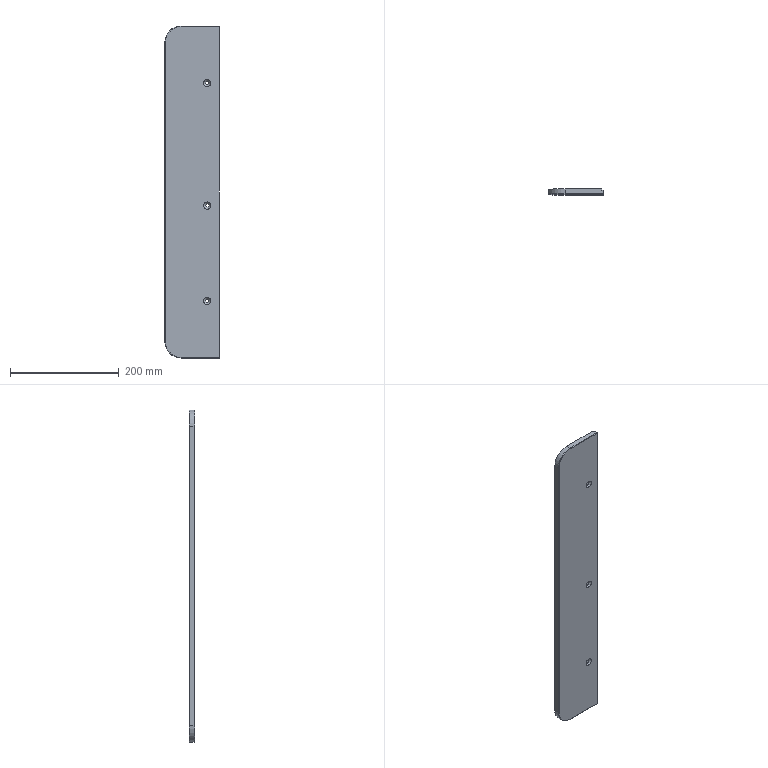Component | SolidWorks | ChainPartTablePlate-1 | 1 solid | 27 faces | box 100 x 10 x 610 mm | volume 601377 mm3 | cylinder 11 | plane 8 | cone 6 | torus 2 | commonest cylinder face diameters 6.6 x6 2 x3 60 x2
build123d program:
from build123d import *

# Parameters (mm, degrees)
SKETCH1_W                                            = 610
SKETCH1_H                                            = 100
BOSS_EXTRUDE1_DEPTH                                  = 10
FILLET1_R                                            = 30
CSK_FOR_M6_HEX_SOCKET_COUNTERSUNK_CAP_SC_D           = 6.6
CSK_FOR_M6_HEX_SOCKET_COUNTERSUNK_CAP_SC_CSINK_D     = 13.6
CSK_FOR_M6_HEX_SOCKET_COUNTERSUNK_CAP_SC_CSINK_ANGLE = 90
SKETCH4_W                                            = 610
SKETCH4_H                                            = 2.5
CUT_EXTRUDE1_DEPTH                                   = 2
FILLET4_R                                            = 1


with BuildPart() as part:
    # Sketch1 → Boss-Extrude1 (new body)
    with BuildSketch(Plane.XY):
        Rectangle(SKETCH1_W, SKETCH1_H)
    extrude(amount=BOSS_EXTRUDE1_DEPTH)

    # Fillet1
    fillet1_edges = [part.edges().sort_by_distance(p)[0] for p in [
        (305, -50, 5),
        (-305, -50, 5),
    ]]
    fillet(fillet1_edges, radius=FILLET1_R)

    # CSK for M6 Hex Socket Countersunk Cap Sc (through all)
    with Locations(Plane.XY.offset(10)):
        with Locations((-200, 28), (200, 28), (25, 28)):
            CounterSinkHole(CSK_FOR_M6_HEX_SOCKET_COUNTERSUNK_CAP_SC_D / 2, CSK_FOR_M6_HEX_SOCKET_COUNTERSUNK_CAP_SC_CSINK_D / 2, counter_sink_angle=CSK_FOR_M6_HEX_SOCKET_COUNTERSUNK_CAP_SC_CSINK_ANGLE)

    # Sketch4 → Cut-Extrude1 (cut)
    with BuildSketch(Plane(origin=(0, 0, 0), x_dir=(-1, 0, 0), z_dir=(0, 0, -1))):
        with Locations((0, 48.75)):
            Rectangle(SKETCH4_W, SKETCH4_H)
    extrude(amount=-CUT_EXTRUDE1_DEPTH, mode=Mode.SUBTRACT)

    # Fillet4
    fillet4_edges = [part.edges().sort_by_distance(p)[0] for p in [
        (-305, 15, 10),
        (0, -50, 10),
        (305, 15, 10),
        (296.213, -41.213, 10),
        (-296.213, -41.213, 10),
    ]]
    fillet(fillet4_edges, radius=FILLET4_R)


solid = part.part

# Placed as in the assembly
solid = solid.moved(Location((32.737, -50.063, -352.804), (90, 0, -90)))